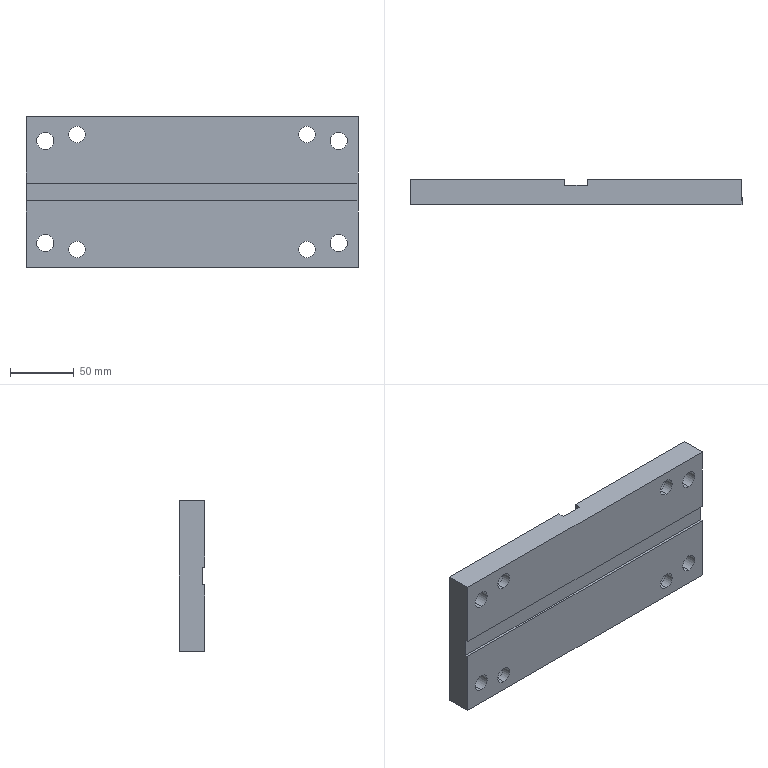Component | SolidWorks | NewTypeCurveBenderReinforcementSeatBase-DoubleWheel-1 | 1 solid | 42 faces | box 260 x 20 x 118 mm | volume 565789 mm3 | cylinder 24 | plane 18 | commonest cylinder face diameters 19 x8 13.5 x8 13 x8
build123d program:
from build123d import *

# Parameters (mm, degrees)
SKETCH1_W           = 260
SKETCH1_H           = 118
BOSS_EXTRUDE1_DEPTH = 20
SKETCH2_R           = 6.75
CUT_EXTRUDE1_DEPTH  = 20
SKETCH3_W           = 18
SKETCH3_H           = 10
CUT_EXTRUDE2_DEPTH  = 177.703
SKETCH4_R           = 6.5
CUT_EXTRUDE3_DEPTH  = 20
SKETCH5_R           = 9.5
CUT_EXTRUDE4_DEPTH  = 13
SKETCH6_W           = 14
SKETCH6_H           = 4
CUT_EXTRUDE5_DEPTH  = 268.359


with BuildPart() as part:
    # Sketch1 → Boss-Extrude1 (new body)
    with BuildSketch(Plane(origin=(0, 0, 0), x_dir=(1, 0, 0), z_dir=(0, 1, 0))):
        Rectangle(SKETCH1_W, SKETCH1_H)
    extrude(amount=BOSS_EXTRUDE1_DEPTH)

    # Sketch2 → Cut-Extrude1 (cut)
    with BuildSketch(Plane(origin=(0, 20, 0), x_dir=(1, 0, 0), z_dir=(0, 1, 0))):
        with Locations(Location((-115, 40, 0), (0, 0, 270))):
            Circle(SKETCH2_R)
        with Locations(Location((115, 40, 0), (0, 0, 90))):
            Circle(SKETCH2_R)
        with Locations(Location((115, -40, 0), (0, 0, 270))):
            Circle(SKETCH2_R)
        with Locations(Location((-115, -40, 0), (0, 0, 90))):
            Circle(SKETCH2_R)
    extrude(amount=-CUT_EXTRUDE1_DEPTH, mode=Mode.SUBTRACT)

    # Sketch3 → Cut-Extrude2 (cut, through all)
    with BuildSketch(Plane.XY.offset(59)):
        Rectangle(SKETCH3_W, SKETCH3_H)
    extrude(amount=-CUT_EXTRUDE2_DEPTH, mode=Mode.SUBTRACT)

    # Sketch4 → Cut-Extrude3 (cut)
    with BuildSketch(Plane.XZ):
        with Locations(Location((-90, 45, 0), (0, 0, 270))):
            Circle(SKETCH4_R)
        with Locations(Location((90, 45, 0), (0, 0, 90))):
            Circle(SKETCH4_R)
        with Locations(Location((90, -45, 0), (0, 0, 270))):
            Circle(SKETCH4_R)
        with Locations(Location((-90, -45, 0), (0, 0, 90))):
            Circle(SKETCH4_R)
    extrude(amount=-CUT_EXTRUDE3_DEPTH, mode=Mode.SUBTRACT)

    # Sketch5 → Cut-Extrude4 (cut)
    with BuildSketch(Plane.XZ):
        with Locations(Location((-90, 45, 0), (0, 0, 270))):
            Circle(SKETCH5_R)
        with Locations(Location((-90, -45, 0), (0, 0, 270))):
            Circle(SKETCH5_R)
        with Locations(Location((90, 45, 0), (0, 0, 270))):
            Circle(SKETCH5_R)
        with Locations(Location((90, -45, 0), (0, 0, 270))):
            Circle(SKETCH5_R)
    extrude(amount=-CUT_EXTRUDE4_DEPTH, mode=Mode.SUBTRACT)

    # Sketch6 → Cut-Extrude5 (cut, through all)
    with BuildSketch(Plane.ZY.offset(130)):
        with Locations((0, 20)):
            Rectangle(SKETCH6_W, SKETCH6_H)
    extrude(amount=-CUT_EXTRUDE5_DEPTH, mode=Mode.SUBTRACT)


solid = part.part

# Placed as in the assembly
solid = solid.moved(Location((0, 20, 0), (180, 0, 0)))